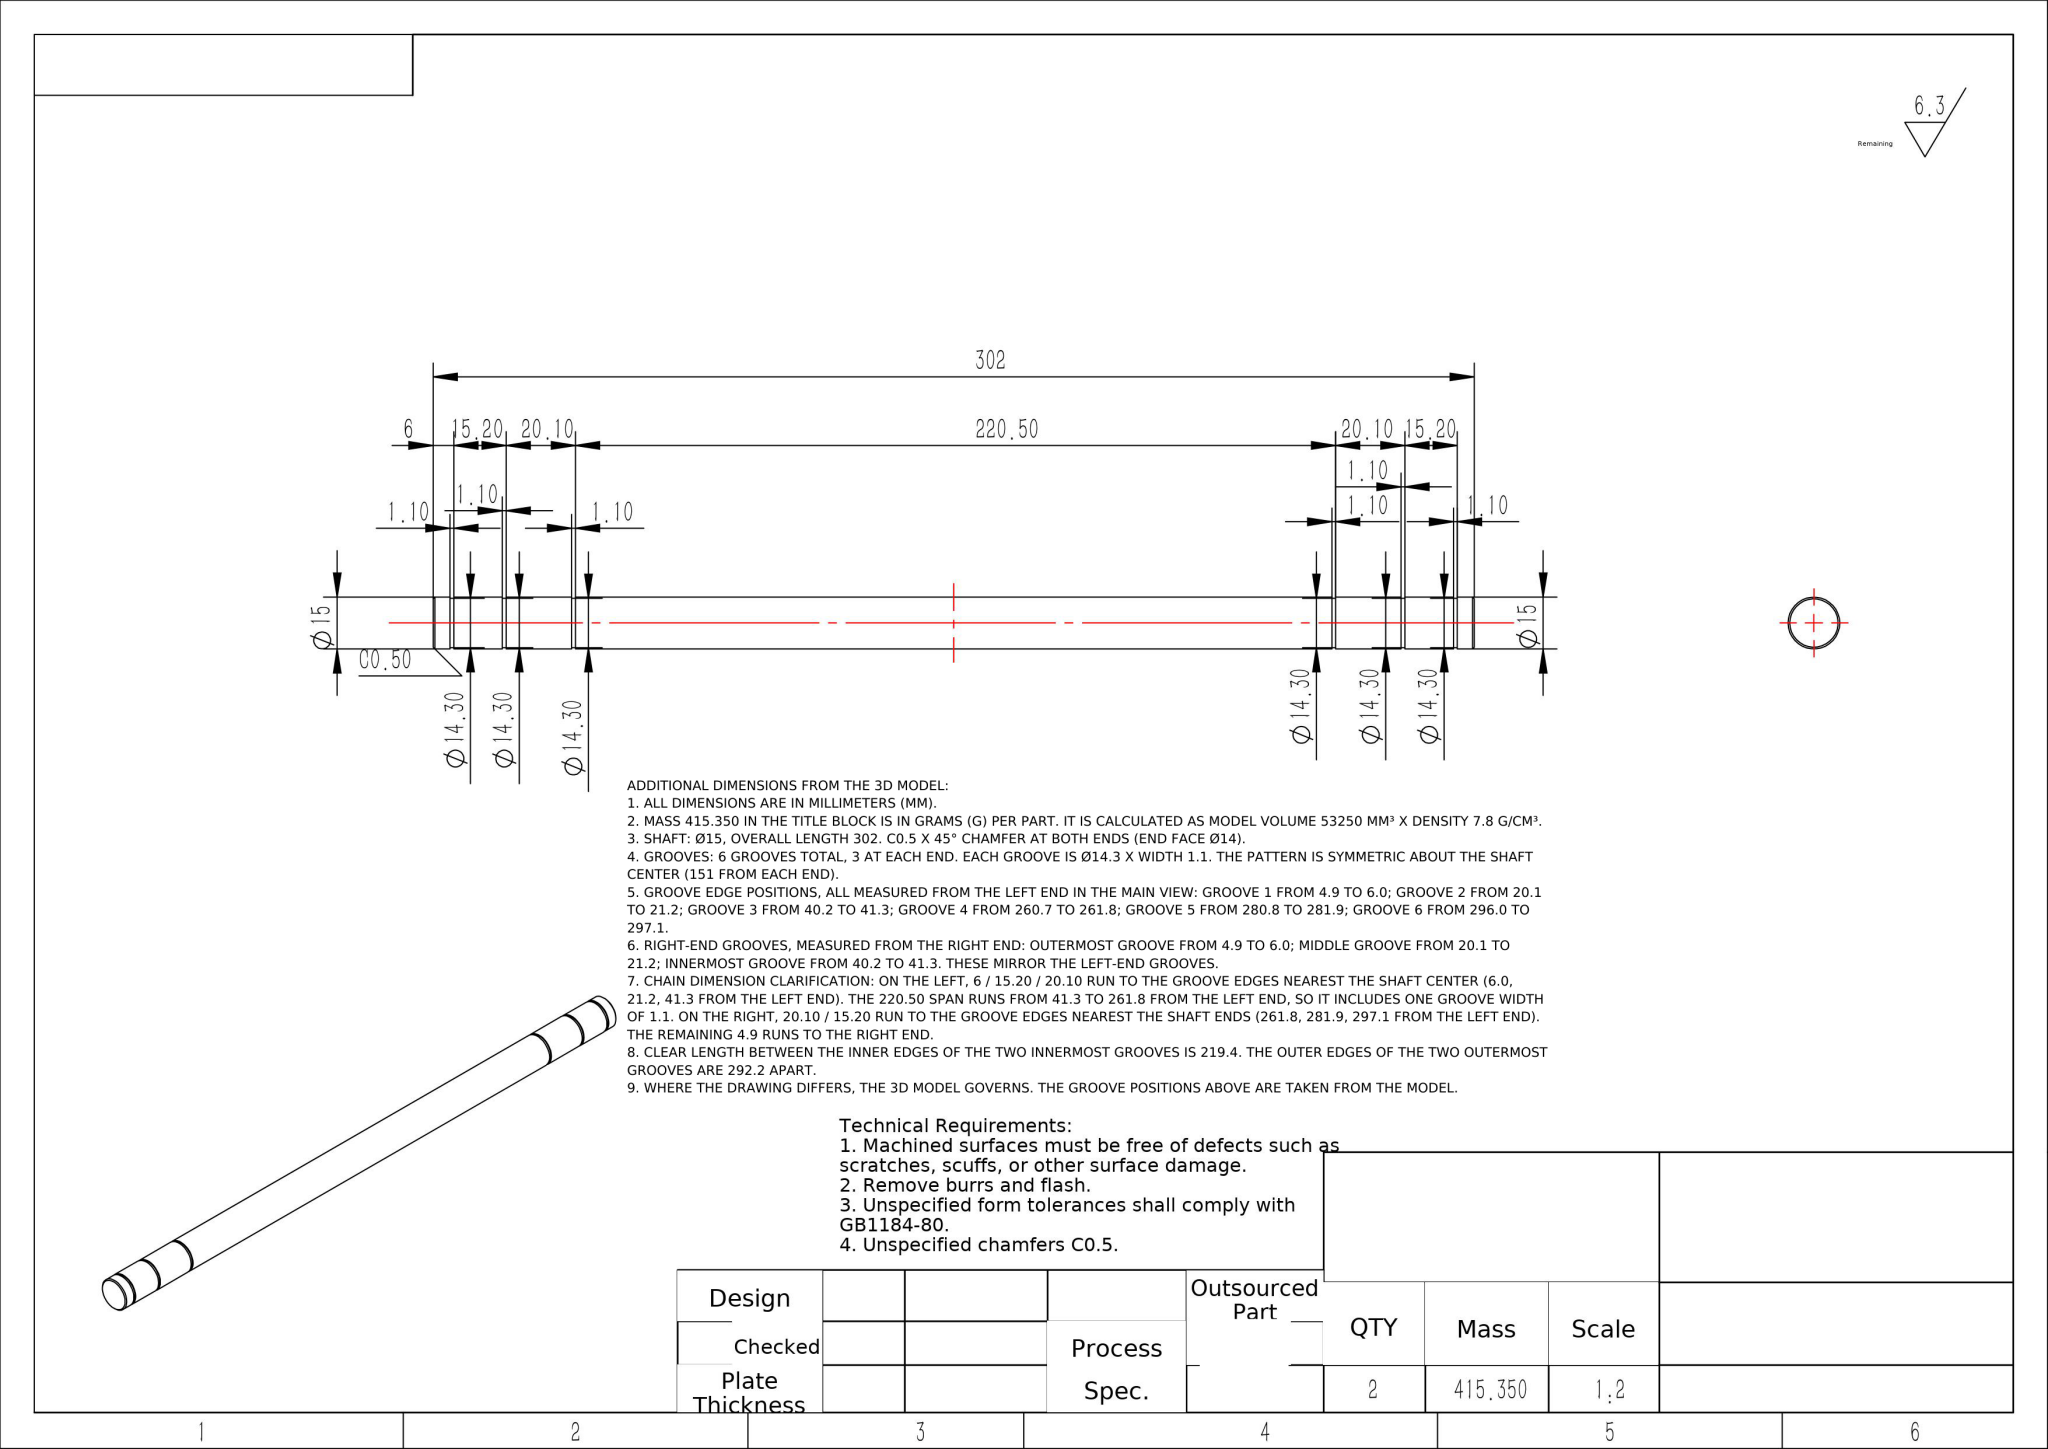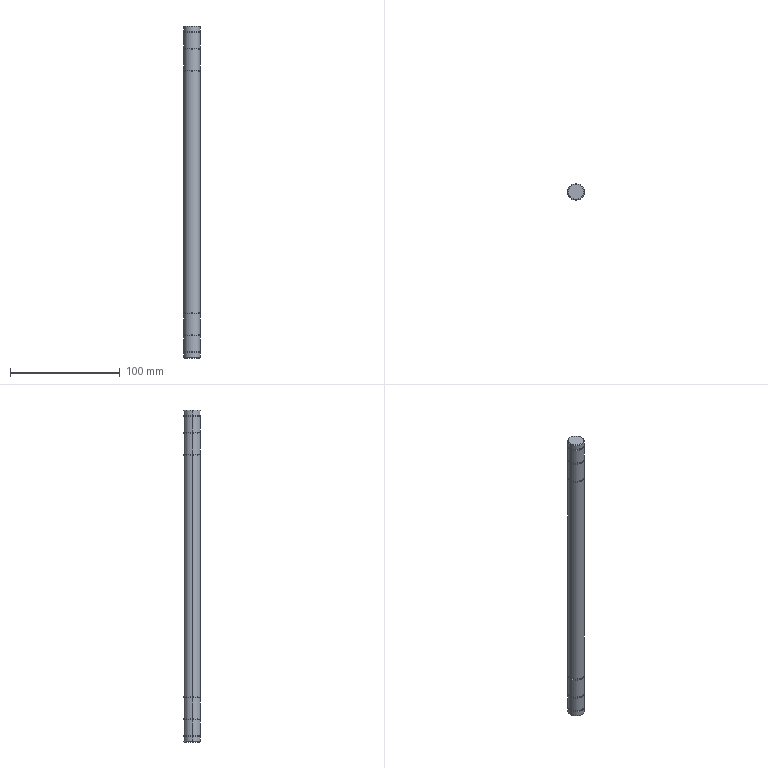Part | NX | mm | 1 solid | 44 faces | box 15 x 15 x 302 mm | volume 53250 mm3 | cylinder 26 | plane 14 | cone 4 | commonest cylinder face diameters 15 x14 14.3 x12